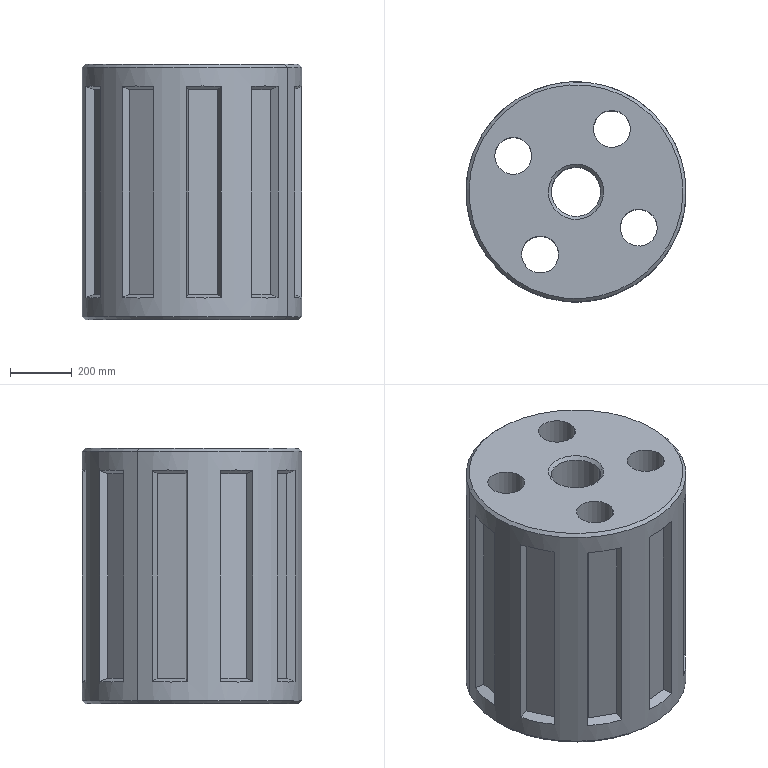Component | SolidWorks | Wheel-1 | 1 solid | 80 faces | volume 256987250 mm3 | plane 52 | cone 16 | cylinder 12 | commonest cylinder face diameters 120 x8 160 x2 715 x2 | material 45